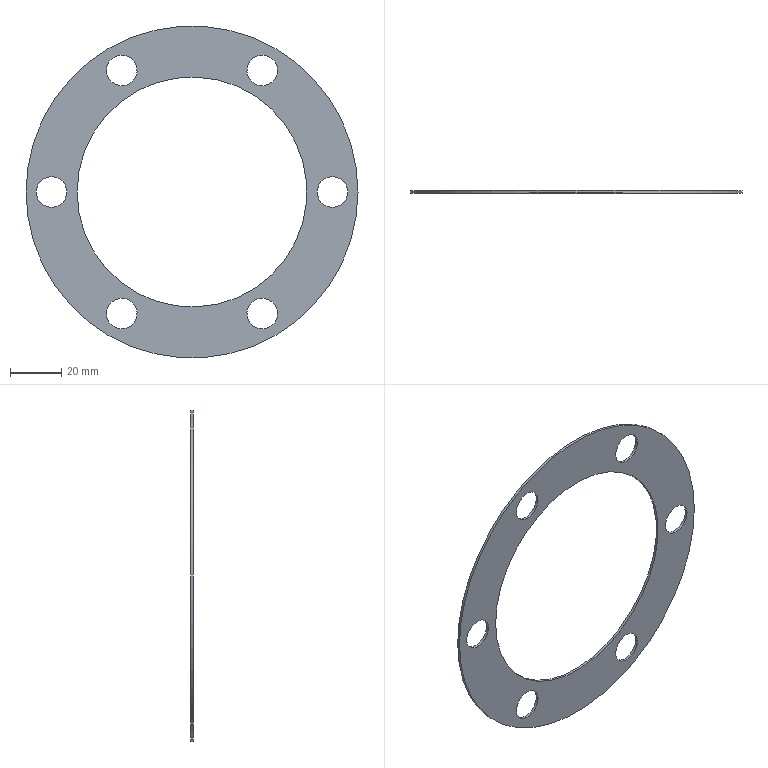Component | NX | T1_SHIM1 | 1 solid | 10 faces | box 130 x 1 x 130 mm | volume 6233 mm3 | cylinder 8 | plane 2 | commonest cylinder face diameters 12 x6 90 x1 130 x1
STEP:
#1=CARTESIAN_POINT('',(0.,0.,0.));
#2=DIRECTION('',(0.,0.,1.));
#3=DIRECTION('',(1.,0.,0.));
#4=AXIS2_PLACEMENT_3D('',#1,#2,#3);
#5=CARTESIAN_POINT('',(-40.,-81.,113.5));
#6=VERTEX_POINT('',#5);
#7=CARTESIAN_POINT('',(5.,-81.,113.5));
#8=DIRECTION('',(0.,1.,0.));
#9=DIRECTION('',(-1.,0.,0.));
#10=AXIS2_PLACEMENT_3D('',#7,#8,#9);
#11=CIRCLE('',#10,45.);
#12=CARTESIAN_POINT('',(5.,-81.,113.5));
#13=DIRECTION('',(0.,-1.,0.));
#14=DIRECTION('',(1.,0.,0.));
#15=AXIS2_PLACEMENT_3D('',#12,#13,#14);
#16=CYLINDRICAL_SURFACE('',#15,45.);
#17=CARTESIAN_POINT('',(9.425,0.));
#18=DIRECTION('',(-1.,0.));
#19=VECTOR('',#18,1.);
#20=LINE('',#17,#19);
#21=(GEOMETRIC_REPRESENTATION_CONTEXT(2)PARAMETRIC_REPRESENTATION_CONTEXT()REPRESENTATION_CONTEXT('',''));
#22=DEFINITIONAL_REPRESENTATION('',(#20),#21);
#23=PCURVE('',#16,#22);
#24=CARTESIAN_POINT('',(-22.5,-81.,113.5));
#25=DIRECTION('',(0.,1.,0.));
#26=DIRECTION('',(-1.,0.,0.));
#27=AXIS2_PLACEMENT_3D('',#24,#25,#26);
#28=PLANE('',#27);
#29=CARTESIAN_POINT('',(-27.5,0.));
#30=DIRECTION('',(1.,0.));
#31=AXIS2_PLACEMENT_2D('',#29,#30);
#32=CIRCLE('',#31,45.);
#33=(GEOMETRIC_REPRESENTATION_CONTEXT(2)PARAMETRIC_REPRESENTATION_CONTEXT()REPRESENTATION_CONTEXT('',''));
#34=DEFINITIONAL_REPRESENTATION('',(#32),#33);
#35=PCURVE('',#28,#34);
#36=SURFACE_CURVE('',#11,(#23,#35),.PCURVE_S1.);
#37=EDGE_CURVE('',#6,#6,#36,.T.);
#38=ORIENTED_EDGE('',*,*,#37,.F.);
#39=CARTESIAN_POINT('',(-40.,-82.,113.5));
#40=VERTEX_POINT('',#39);
#41=CARTESIAN_POINT('',(-40.,-81.,113.5));
#42=CARTESIAN_POINT('',(-40.,-82.,113.5));
#43=B_SPLINE_CURVE_WITH_KNOTS('',1,(#41,#42),.UNSPECIFIED.,.F.,.F.,(2,2),(0.,1.),.PIECEWISE_BEZIER_KNOTS.);
#44=CARTESIAN_POINT('',(9.425,0.));
#45=DIRECTION('',(0.,1.));
#46=VECTOR('',#45,1.);
#47=LINE('',#44,#46);
#48=(GEOMETRIC_REPRESENTATION_CONTEXT(2)PARAMETRIC_REPRESENTATION_CONTEXT()REPRESENTATION_CONTEXT('',''));
#49=DEFINITIONAL_REPRESENTATION('',(#47),#48);
#50=PCURVE('',#16,#49);
#51=CARTESIAN_POINT('',(3.142,0.));
#52=DIRECTION('',(0.,1.));
#53=VECTOR('',#52,1.);
#54=LINE('',#51,#53);
#55=(GEOMETRIC_REPRESENTATION_CONTEXT(2)PARAMETRIC_REPRESENTATION_CONTEXT()REPRESENTATION_CONTEXT('',''));
#56=DEFINITIONAL_REPRESENTATION('',(#54),#55);
#57=PCURVE('',#16,#56);
#58=SEAM_CURVE('',#43,(#50,#57),.PCURVE_S1.);
#59=EDGE_CURVE('',#6,#40,#58,.T.);
#60=ORIENTED_EDGE('',*,*,#59,.T.);
#61=CARTESIAN_POINT('',(5.,-82.,113.5));
#62=DIRECTION('',(0.,1.,0.));
#63=DIRECTION('',(-1.,0.,0.));
#64=AXIS2_PLACEMENT_3D('',#61,#62,#63);
#65=CIRCLE('',#64,45.);
#66=CARTESIAN_POINT('',(9.425,1.));
#67=DIRECTION('',(-1.,0.));
#68=VECTOR('',#67,1.);
#69=LINE('',#66,#68);
#70=(GEOMETRIC_REPRESENTATION_CONTEXT(2)PARAMETRIC_REPRESENTATION_CONTEXT()REPRESENTATION_CONTEXT('',''));
#71=DEFINITIONAL_REPRESENTATION('',(#69),#70);
#72=PCURVE('',#16,#71);
#73=CARTESIAN_POINT('',(-22.5,-82.,113.5));
#74=DIRECTION('',(0.,1.,0.));
#75=DIRECTION('',(-1.,0.,0.));
#76=AXIS2_PLACEMENT_3D('',#73,#74,#75);
#77=PLANE('',#76);
#78=CARTESIAN_POINT('',(-27.5,0.));
#79=DIRECTION('',(1.,0.));
#80=AXIS2_PLACEMENT_2D('',#78,#79);
#81=CIRCLE('',#80,45.);
#82=(GEOMETRIC_REPRESENTATION_CONTEXT(2)PARAMETRIC_REPRESENTATION_CONTEXT()REPRESENTATION_CONTEXT('',''));
#83=DEFINITIONAL_REPRESENTATION('',(#81),#82);
#84=PCURVE('',#77,#83);
#85=SURFACE_CURVE('',#65,(#72,#84),.PCURVE_S1.);
#86=EDGE_CURVE('',#40,#40,#85,.T.);
#87=ORIENTED_EDGE('',*,*,#86,.T.);
#88=ORIENTED_EDGE('',*,*,#59,.F.);
#89=EDGE_LOOP('',(#38,#60,#87,#88));
#90=FACE_BOUND('',#89,.F.);
#91=ADVANCED_FACE('',(#90),#16,.F.);
#92=CARTESIAN_POINT('',(35.5,-81.,60.672));
#93=VERTEX_POINT('',#92);
#94=CARTESIAN_POINT('',(32.5,-81.,65.869));
#95=DIRECTION('',(0.,1.,0.));
#96=DIRECTION('',(0.5,0.,-0.866));
#97=AXIS2_PLACEMENT_3D('',#94,#95,#96);
#98=CIRCLE('',#97,6.);
#99=CARTESIAN_POINT('',(32.5,-81.,65.869));
#100=DIRECTION('',(0.,-1.,0.));
#101=DIRECTION('',(1.,0.,0.));
#102=AXIS2_PLACEMENT_3D('',#99,#100,#101);
#103=CYLINDRICAL_SURFACE('',#102,6.);
#104=CARTESIAN_POINT('',(11.519,0.));
#105=DIRECTION('',(-1.,0.));
#106=VECTOR('',#105,1.);
#107=LINE('',#104,#106);
#108=(GEOMETRIC_REPRESENTATION_CONTEXT(2)PARAMETRIC_REPRESENTATION_CONTEXT()REPRESENTATION_CONTEXT('',''));
#109=DEFINITIONAL_REPRESENTATION('',(#107),#108);
#110=PCURVE('',#103,#109);
#111=CARTESIAN_POINT('',(-55.,-47.631));
#112=DIRECTION('',(-0.5,-0.866));
#113=AXIS2_PLACEMENT_2D('',#111,#112);
#114=CIRCLE('',#113,6.);
#115=(GEOMETRIC_REPRESENTATION_CONTEXT(2)PARAMETRIC_REPRESENTATION_CONTEXT()REPRESENTATION_CONTEXT('',''));
#116=DEFINITIONAL_REPRESENTATION('',(#114),#115);
#117=PCURVE('',#28,#116);
#118=SURFACE_CURVE('',#98,(#110,#117),.PCURVE_S1.);
#119=EDGE_CURVE('',#93,#93,#118,.T.);
#120=ORIENTED_EDGE('',*,*,#119,.F.);
#121=CARTESIAN_POINT('',(35.5,-82.,60.672));
#122=VERTEX_POINT('',#121);
#123=CARTESIAN_POINT('',(35.5,-81.,60.672));
#124=CARTESIAN_POINT('',(35.5,-82.,60.672));
#125=B_SPLINE_CURVE_WITH_KNOTS('',1,(#123,#124),.UNSPECIFIED.,.F.,.F.,(2,2),(0.,1.),.PIECEWISE_BEZIER_KNOTS.);
#126=CARTESIAN_POINT('',(11.519,0.));
#127=DIRECTION('',(0.,1.));
#128=VECTOR('',#127,1.);
#129=LINE('',#126,#128);
#130=(GEOMETRIC_REPRESENTATION_CONTEXT(2)PARAMETRIC_REPRESENTATION_CONTEXT()REPRESENTATION_CONTEXT('',''));
#131=DEFINITIONAL_REPRESENTATION('',(#129),#130);
#132=PCURVE('',#103,#131);
#133=CARTESIAN_POINT('',(5.236,0.));
#134=DIRECTION('',(0.,1.));
#135=VECTOR('',#134,1.);
#136=LINE('',#133,#135);
#137=(GEOMETRIC_REPRESENTATION_CONTEXT(2)PARAMETRIC_REPRESENTATION_CONTEXT()REPRESENTATION_CONTEXT('',''));
#138=DEFINITIONAL_REPRESENTATION('',(#136),#137);
#139=PCURVE('',#103,#138);
#140=SEAM_CURVE('',#125,(#132,#139),.PCURVE_S1.);
#141=EDGE_CURVE('',#93,#122,#140,.T.);
#142=ORIENTED_EDGE('',*,*,#141,.T.);
#143=CARTESIAN_POINT('',(32.5,-82.,65.869));
#144=DIRECTION('',(0.,1.,0.));
#145=DIRECTION('',(0.5,0.,-0.866));
#146=AXIS2_PLACEMENT_3D('',#143,#144,#145);
#147=CIRCLE('',#146,6.);
#148=CARTESIAN_POINT('',(11.519,1.));
#149=DIRECTION('',(-1.,0.));
#150=VECTOR('',#149,1.);
#151=LINE('',#148,#150);
#152=(GEOMETRIC_REPRESENTATION_CONTEXT(2)PARAMETRIC_REPRESENTATION_CONTEXT()REPRESENTATION_CONTEXT('',''));
#153=DEFINITIONAL_REPRESENTATION('',(#151),#152);
#154=PCURVE('',#103,#153);
#155=CARTESIAN_POINT('',(-55.,-47.631));
#156=DIRECTION('',(-0.5,-0.866));
#157=AXIS2_PLACEMENT_2D('',#155,#156);
#158=CIRCLE('',#157,6.);
#159=(GEOMETRIC_REPRESENTATION_CONTEXT(2)PARAMETRIC_REPRESENTATION_CONTEXT()REPRESENTATION_CONTEXT('',''));
#160=DEFINITIONAL_REPRESENTATION('',(#158),#159);
#161=PCURVE('',#77,#160);
#162=SURFACE_CURVE('',#147,(#154,#161),.PCURVE_S1.);
#163=EDGE_CURVE('',#122,#122,#162,.T.);
#164=ORIENTED_EDGE('',*,*,#163,.T.);
#165=ORIENTED_EDGE('',*,*,#141,.F.);
#166=EDGE_LOOP('',(#120,#142,#164,#165));
#167=FACE_BOUND('',#166,.F.);
#168=ADVANCED_FACE('',(#167),#103,.F.);
#169=CARTESIAN_POINT('',(35.5,-81.,166.328));
#170=VERTEX_POINT('',#169);
#171=CARTESIAN_POINT('',(32.5,-81.,161.131));
#172=DIRECTION('',(0.,1.,0.));
#173=DIRECTION('',(0.5,0.,0.866));
#174=AXIS2_PLACEMENT_3D('',#171,#172,#173);
#175=CIRCLE('',#174,6.);
#176=CARTESIAN_POINT('',(32.5,-81.,161.131));
#177=DIRECTION('',(0.,-1.,0.));
#178=DIRECTION('',(1.,0.,0.));
#179=AXIS2_PLACEMENT_3D('',#176,#177,#178);
#180=CYLINDRICAL_SURFACE('',#179,6.);
#181=CARTESIAN_POINT('',(7.33,0.));
#182=DIRECTION('',(-1.,0.));
#183=VECTOR('',#182,1.);
#184=LINE('',#181,#183);
#185=(GEOMETRIC_REPRESENTATION_CONTEXT(2)PARAMETRIC_REPRESENTATION_CONTEXT()REPRESENTATION_CONTEXT('',''));
#186=DEFINITIONAL_REPRESENTATION('',(#184),#185);
#187=PCURVE('',#180,#186);
#188=CARTESIAN_POINT('',(-55.,47.631));
#189=DIRECTION('',(-0.5,0.866));
#190=AXIS2_PLACEMENT_2D('',#188,#189);
#191=CIRCLE('',#190,6.);
#192=(GEOMETRIC_REPRESENTATION_CONTEXT(2)PARAMETRIC_REPRESENTATION_CONTEXT()REPRESENTATION_CONTEXT('',''));
#193=DEFINITIONAL_REPRESENTATION('',(#191),#192);
#194=PCURVE('',#28,#193);
#195=SURFACE_CURVE('',#175,(#187,#194),.PCURVE_S1.);
#196=EDGE_CURVE('',#170,#170,#195,.T.);
#197=ORIENTED_EDGE('',*,*,#196,.F.);
#198=CARTESIAN_POINT('',(35.5,-82.,166.328));
#199=VERTEX_POINT('',#198);
#200=CARTESIAN_POINT('',(35.5,-81.,166.328));
#201=CARTESIAN_POINT('',(35.5,-82.,166.328));
#202=B_SPLINE_CURVE_WITH_KNOTS('',1,(#200,#201),.UNSPECIFIED.,.F.,.F.,(2,2),(0.,1.),.PIECEWISE_BEZIER_KNOTS.);
#203=CARTESIAN_POINT('',(7.33,0.));
#204=DIRECTION('',(0.,1.));
#205=VECTOR('',#204,1.);
#206=LINE('',#203,#205);
#207=(GEOMETRIC_REPRESENTATION_CONTEXT(2)PARAMETRIC_REPRESENTATION_CONTEXT()REPRESENTATION_CONTEXT('',''));
#208=DEFINITIONAL_REPRESENTATION('',(#206),#207);
#209=PCURVE('',#180,#208);
#210=CARTESIAN_POINT('',(1.047,0.));
#211=DIRECTION('',(0.,1.));
#212=VECTOR('',#211,1.);
#213=LINE('',#210,#212);
#214=(GEOMETRIC_REPRESENTATION_CONTEXT(2)PARAMETRIC_REPRESENTATION_CONTEXT()REPRESENTATION_CONTEXT('',''));
#215=DEFINITIONAL_REPRESENTATION('',(#213),#214);
#216=PCURVE('',#180,#215);
#217=SEAM_CURVE('',#202,(#209,#216),.PCURVE_S1.);
#218=EDGE_CURVE('',#170,#199,#217,.T.);
#219=ORIENTED_EDGE('',*,*,#218,.T.);
#220=CARTESIAN_POINT('',(32.5,-82.,161.131));
#221=DIRECTION('',(0.,1.,0.));
#222=DIRECTION('',(0.5,0.,0.866));
#223=AXIS2_PLACEMENT_3D('',#220,#221,#222);
#224=CIRCLE('',#223,6.);
#225=CARTESIAN_POINT('',(7.33,1.));
#226=DIRECTION('',(-1.,0.));
#227=VECTOR('',#226,1.);
#228=LINE('',#225,#227);
#229=(GEOMETRIC_REPRESENTATION_CONTEXT(2)PARAMETRIC_REPRESENTATION_CONTEXT()REPRESENTATION_CONTEXT('',''));
#230=DEFINITIONAL_REPRESENTATION('',(#228),#229);
#231=PCURVE('',#180,#230);
#232=CARTESIAN_POINT('',(-55.,47.631));
#233=DIRECTION('',(-0.5,0.866));
#234=AXIS2_PLACEMENT_2D('',#232,#233);
#235=CIRCLE('',#234,6.);
#236=(GEOMETRIC_REPRESENTATION_CONTEXT(2)PARAMETRIC_REPRESENTATION_CONTEXT()REPRESENTATION_CONTEXT('',''));
#237=DEFINITIONAL_REPRESENTATION('',(#235),#236);
#238=PCURVE('',#77,#237);
#239=SURFACE_CURVE('',#224,(#231,#238),.PCURVE_S1.);
#240=EDGE_CURVE('',#199,#199,#239,.T.);
#241=ORIENTED_EDGE('',*,*,#240,.T.);
#242=ORIENTED_EDGE('',*,*,#218,.F.);
#243=EDGE_LOOP('',(#197,#219,#241,#242));
#244=FACE_BOUND('',#243,.F.);
#245=ADVANCED_FACE('',(#244),#180,.F.);
#246=CARTESIAN_POINT('',(-25.5,-81.,60.672));
#247=VERTEX_POINT('',#246);
#248=CARTESIAN_POINT('',(-22.5,-81.,65.869));
#249=DIRECTION('',(0.,1.,0.));
#250=DIRECTION('',(-0.5,0.,-0.866));
#251=AXIS2_PLACEMENT_3D('',#248,#249,#250);
#252=CIRCLE('',#251,6.);
#253=CARTESIAN_POINT('',(-22.5,-81.,65.869));
#254=DIRECTION('',(0.,-1.,0.));
#255=DIRECTION('',(1.,0.,0.));
#256=AXIS2_PLACEMENT_3D('',#253,#254,#255);
#257=CYLINDRICAL_SURFACE('',#256,6.);
#258=CARTESIAN_POINT('',(10.472,0.));
#259=DIRECTION('',(-1.,0.));
#260=VECTOR('',#259,1.);
#261=LINE('',#258,#260);
#262=(GEOMETRIC_REPRESENTATION_CONTEXT(2)PARAMETRIC_REPRESENTATION_CONTEXT()REPRESENTATION_CONTEXT('',''));
#263=DEFINITIONAL_REPRESENTATION('',(#261),#262);
#264=PCURVE('',#257,#263);
#265=CARTESIAN_POINT('',(-0.,-47.631));
#266=DIRECTION('',(0.5,-0.866));
#267=AXIS2_PLACEMENT_2D('',#265,#266);
#268=CIRCLE('',#267,6.);
#269=(GEOMETRIC_REPRESENTATION_CONTEXT(2)PARAMETRIC_REPRESENTATION_CONTEXT()REPRESENTATION_CONTEXT('',''));
#270=DEFINITIONAL_REPRESENTATION('',(#268),#269);
#271=PCURVE('',#28,#270);
#272=SURFACE_CURVE('',#252,(#264,#271),.PCURVE_S1.);
#273=EDGE_CURVE('',#247,#247,#272,.T.);
#274=ORIENTED_EDGE('',*,*,#273,.F.);
#275=CARTESIAN_POINT('',(-25.5,-82.,60.672));
#276=VERTEX_POINT('',#275);
#277=CARTESIAN_POINT('',(-25.5,-81.,60.672));
#278=CARTESIAN_POINT('',(-25.5,-82.,60.672));
#279=B_SPLINE_CURVE_WITH_KNOTS('',1,(#277,#278),.UNSPECIFIED.,.F.,.F.,(2,2),(0.,1.),.PIECEWISE_BEZIER_KNOTS.);
#280=CARTESIAN_POINT('',(10.472,0.));
#281=DIRECTION('',(0.,1.));
#282=VECTOR('',#281,1.);
#283=LINE('',#280,#282);
#284=(GEOMETRIC_REPRESENTATION_CONTEXT(2)PARAMETRIC_REPRESENTATION_CONTEXT()REPRESENTATION_CONTEXT('',''));
#285=DEFINITIONAL_REPRESENTATION('',(#283),#284);
#286=PCURVE('',#257,#285);
#287=CARTESIAN_POINT('',(4.189,0.));
#288=DIRECTION('',(0.,1.));
#289=VECTOR('',#288,1.);
#290=LINE('',#287,#289);
#291=(GEOMETRIC_REPRESENTATION_CONTEXT(2)PARAMETRIC_REPRESENTATION_CONTEXT()REPRESENTATION_CONTEXT('',''));
#292=DEFINITIONAL_REPRESENTATION('',(#290),#291);
#293=PCURVE('',#257,#292);
#294=SEAM_CURVE('',#279,(#286,#293),.PCURVE_S1.);
#295=EDGE_CURVE('',#247,#276,#294,.T.);
#296=ORIENTED_EDGE('',*,*,#295,.T.);
#297=CARTESIAN_POINT('',(-22.5,-82.,65.869));
#298=DIRECTION('',(0.,1.,0.));
#299=DIRECTION('',(-0.5,0.,-0.866));
#300=AXIS2_PLACEMENT_3D('',#297,#298,#299);
#301=CIRCLE('',#300,6.);
#302=CARTESIAN_POINT('',(10.472,1.));
#303=DIRECTION('',(-1.,0.));
#304=VECTOR('',#303,1.);
#305=LINE('',#302,#304);
#306=(GEOMETRIC_REPRESENTATION_CONTEXT(2)PARAMETRIC_REPRESENTATION_CONTEXT()REPRESENTATION_CONTEXT('',''));
#307=DEFINITIONAL_REPRESENTATION('',(#305),#306);
#308=PCURVE('',#257,#307);
#309=CARTESIAN_POINT('',(-0.,-47.631));
#310=DIRECTION('',(0.5,-0.866));
#311=AXIS2_PLACEMENT_2D('',#309,#310);
#312=CIRCLE('',#311,6.);
#313=(GEOMETRIC_REPRESENTATION_CONTEXT(2)PARAMETRIC_REPRESENTATION_CONTEXT()REPRESENTATION_CONTEXT('',''));
#314=DEFINITIONAL_REPRESENTATION('',(#312),#313);
#315=PCURVE('',#77,#314);
#316=SURFACE_CURVE('',#301,(#308,#315),.PCURVE_S1.);
#317=EDGE_CURVE('',#276,#276,#316,.T.);
#318=ORIENTED_EDGE('',*,*,#317,.T.);
#319=ORIENTED_EDGE('',*,*,#295,.F.);
#320=EDGE_LOOP('',(#274,#296,#318,#319));
#321=FACE_BOUND('',#320,.F.);
#322=ADVANCED_FACE('',(#321),#257,.F.);
#323=CARTESIAN_POINT('',(-25.5,-81.,166.328));
#324=VERTEX_POINT('',#323);
#325=CARTESIAN_POINT('',(-22.5,-81.,161.131));
#326=DIRECTION('',(0.,1.,0.));
#327=DIRECTION('',(-0.5,0.,0.866));
#328=AXIS2_PLACEMENT_3D('',#325,#326,#327);
#329=CIRCLE('',#328,6.);
#330=CARTESIAN_POINT('',(-22.5,-81.,161.131));
#331=DIRECTION('',(0.,-1.,0.));
#332=DIRECTION('',(1.,0.,0.));
#333=AXIS2_PLACEMENT_3D('',#330,#331,#332);
#334=CYLINDRICAL_SURFACE('',#333,6.);
#335=CARTESIAN_POINT('',(8.378,0.));
#336=DIRECTION('',(-1.,0.));
#337=VECTOR('',#336,1.);
#338=LINE('',#335,#337);
#339=(GEOMETRIC_REPRESENTATION_CONTEXT(2)PARAMETRIC_REPRESENTATION_CONTEXT()REPRESENTATION_CONTEXT('',''));
#340=DEFINITIONAL_REPRESENTATION('',(#338),#339);
#341=PCURVE('',#334,#340);
#342=CARTESIAN_POINT('',(0.,47.631));
#343=DIRECTION('',(0.5,0.866));
#344=AXIS2_PLACEMENT_2D('',#342,#343);
#345=CIRCLE('',#344,6.);
#346=(GEOMETRIC_REPRESENTATION_CONTEXT(2)PARAMETRIC_REPRESENTATION_CONTEXT()REPRESENTATION_CONTEXT('',''));
#347=DEFINITIONAL_REPRESENTATION('',(#345),#346);
#348=PCURVE('',#28,#347);
#349=SURFACE_CURVE('',#329,(#341,#348),.PCURVE_S1.);
#350=EDGE_CURVE('',#324,#324,#349,.T.);
#351=ORIENTED_EDGE('',*,*,#350,.F.);
#352=CARTESIAN_POINT('',(-25.5,-82.,166.328));
#353=VERTEX_POINT('',#352);
#354=CARTESIAN_POINT('',(-25.5,-81.,166.328));
#355=CARTESIAN_POINT('',(-25.5,-82.,166.328));
#356=B_SPLINE_CURVE_WITH_KNOTS('',1,(#354,#355),.UNSPECIFIED.,.F.,.F.,(2,2),(0.,1.),.PIECEWISE_BEZIER_KNOTS.);
#357=CARTESIAN_POINT('',(8.378,0.));
#358=DIRECTION('',(0.,1.));
#359=VECTOR('',#358,1.);
#360=LINE('',#357,#359);
#361=(GEOMETRIC_REPRESENTATION_CONTEXT(2)PARAMETRIC_REPRESENTATION_CONTEXT()REPRESENTATION_CONTEXT('',''));
#362=DEFINITIONAL_REPRESENTATION('',(#360),#361);
#363=PCURVE('',#334,#362);
#364=CARTESIAN_POINT('',(2.094,0.));
#365=DIRECTION('',(0.,1.));
#366=VECTOR('',#365,1.);
#367=LINE('',#364,#366);
#368=(GEOMETRIC_REPRESENTATION_CONTEXT(2)PARAMETRIC_REPRESENTATION_CONTEXT()REPRESENTATION_CONTEXT('',''));
#369=DEFINITIONAL_REPRESENTATION('',(#367),#368);
#370=PCURVE('',#334,#369);
#371=SEAM_CURVE('',#356,(#363,#370),.PCURVE_S1.);
#372=EDGE_CURVE('',#324,#353,#371,.T.);
#373=ORIENTED_EDGE('',*,*,#372,.T.);
#374=CARTESIAN_POINT('',(-22.5,-82.,161.131));
#375=DIRECTION('',(0.,1.,0.));
#376=DIRECTION('',(-0.5,0.,0.866));
#377=AXIS2_PLACEMENT_3D('',#374,#375,#376);
#378=CIRCLE('',#377,6.);
#379=CARTESIAN_POINT('',(8.378,1.));
#380=DIRECTION('',(-1.,0.));
#381=VECTOR('',#380,1.);
#382=LINE('',#379,#381);
#383=(GEOMETRIC_REPRESENTATION_CONTEXT(2)PARAMETRIC_REPRESENTATION_CONTEXT()REPRESENTATION_CONTEXT('',''));
#384=DEFINITIONAL_REPRESENTATION('',(#382),#383);
#385=PCURVE('',#334,#384);
#386=CARTESIAN_POINT('',(0.,47.631));
#387=DIRECTION('',(0.5,0.866));
#388=AXIS2_PLACEMENT_2D('',#386,#387);
#389=CIRCLE('',#388,6.);
#390=(GEOMETRIC_REPRESENTATION_CONTEXT(2)PARAMETRIC_REPRESENTATION_CONTEXT()REPRESENTATION_CONTEXT('',''));
#391=DEFINITIONAL_REPRESENTATION('',(#389),#390);
#392=PCURVE('',#77,#391);
#393=SURFACE_CURVE('',#378,(#385,#392),.PCURVE_S1.);
#394=EDGE_CURVE('',#353,#353,#393,.T.);
#395=ORIENTED_EDGE('',*,*,#394,.T.);
#396=ORIENTED_EDGE('',*,*,#372,.F.);
#397=EDGE_LOOP('',(#351,#373,#395,#396));
#398=FACE_BOUND('',#397,.F.);
#399=ADVANCED_FACE('',(#398),#334,.F.);
#400=CARTESIAN_POINT('',(-56.,-81.,113.5));
#401=VERTEX_POINT('',#400);
#402=CARTESIAN_POINT('',(-50.,-81.,113.5));
#403=DIRECTION('',(0.,1.,0.));
#404=DIRECTION('',(-1.,0.,0.));
#405=AXIS2_PLACEMENT_3D('',#402,#403,#404);
#406=CIRCLE('',#405,6.);
#407=CARTESIAN_POINT('',(-50.,-81.,113.5));
#408=DIRECTION('',(0.,-1.,0.));
#409=DIRECTION('',(1.,0.,0.));
#410=AXIS2_PLACEMENT_3D('',#407,#408,#409);
#411=CYLINDRICAL_SURFACE('',#410,6.);
#412=CARTESIAN_POINT('',(9.425,0.));
#413=DIRECTION('',(-1.,0.));
#414=VECTOR('',#413,1.);
#415=LINE('',#412,#414);
#416=(GEOMETRIC_REPRESENTATION_CONTEXT(2)PARAMETRIC_REPRESENTATION_CONTEXT()REPRESENTATION_CONTEXT('',''));
#417=DEFINITIONAL_REPRESENTATION('',(#415),#416);
#418=PCURVE('',#411,#417);
#419=CARTESIAN_POINT('',(27.5,0.));
#420=DIRECTION('',(1.,0.));
#421=AXIS2_PLACEMENT_2D('',#419,#420);
#422=CIRCLE('',#421,6.);
#423=(GEOMETRIC_REPRESENTATION_CONTEXT(2)PARAMETRIC_REPRESENTATION_CONTEXT()REPRESENTATION_CONTEXT('',''));
#424=DEFINITIONAL_REPRESENTATION('',(#422),#423);
#425=PCURVE('',#28,#424);
#426=SURFACE_CURVE('',#406,(#418,#425),.PCURVE_S1.);
#427=EDGE_CURVE('',#401,#401,#426,.T.);
#428=ORIENTED_EDGE('',*,*,#427,.F.);
#429=CARTESIAN_POINT('',(-56.,-82.,113.5));
#430=VERTEX_POINT('',#429);
#431=CARTESIAN_POINT('',(-56.,-81.,113.5));
#432=CARTESIAN_POINT('',(-56.,-82.,113.5));
#433=B_SPLINE_CURVE_WITH_KNOTS('',1,(#431,#432),.UNSPECIFIED.,.F.,.F.,(2,2),(0.,1.),.PIECEWISE_BEZIER_KNOTS.);
#434=CARTESIAN_POINT('',(9.425,0.));
#435=DIRECTION('',(0.,1.));
#436=VECTOR('',#435,1.);
#437=LINE('',#434,#436);
#438=(GEOMETRIC_REPRESENTATION_CONTEXT(2)PARAMETRIC_REPRESENTATION_CONTEXT()REPRESENTATION_CONTEXT('',''));
#439=DEFINITIONAL_REPRESENTATION('',(#437),#438);
#440=PCURVE('',#411,#439);
#441=CARTESIAN_POINT('',(3.142,0.));
#442=DIRECTION('',(0.,1.));
#443=VECTOR('',#442,1.);
#444=LINE('',#441,#443);
#445=(GEOMETRIC_REPRESENTATION_CONTEXT(2)PARAMETRIC_REPRESENTATION_CONTEXT()REPRESENTATION_CONTEXT('',''));
#446=DEFINITIONAL_REPRESENTATION('',(#444),#445);
#447=PCURVE('',#411,#446);
#448=SEAM_CURVE('',#433,(#440,#447),.PCURVE_S1.);
#449=EDGE_CURVE('',#401,#430,#448,.T.);
#450=ORIENTED_EDGE('',*,*,#449,.T.);
#451=CARTESIAN_POINT('',(-50.,-82.,113.5));
#452=DIRECTION('',(0.,1.,0.));
#453=DIRECTION('',(-1.,0.,0.));
#454=AXIS2_PLACEMENT_3D('',#451,#452,#453);
#455=CIRCLE('',#454,6.);
#456=CARTESIAN_POINT('',(9.425,1.));
#457=DIRECTION('',(-1.,0.));
#458=VECTOR('',#457,1.);
#459=LINE('',#456,#458);
#460=(GEOMETRIC_REPRESENTATION_CONTEXT(2)PARAMETRIC_REPRESENTATION_CONTEXT()REPRESENTATION_CONTEXT('',''));
#461=DEFINITIONAL_REPRESENTATION('',(#459),#460);
#462=PCURVE('',#411,#461);
#463=CARTESIAN_POINT('',(27.5,0.));
#464=DIRECTION('',(1.,0.));
#465=AXIS2_PLACEMENT_2D('',#463,#464);
#466=CIRCLE('',#465,6.);
#467=(GEOMETRIC_REPRESENTATION_CONTEXT(2)PARAMETRIC_REPRESENTATION_CONTEXT()REPRESENTATION_CONTEXT('',''));
#468=DEFINITIONAL_REPRESENTATION('',(#466),#467);
#469=PCURVE('',#77,#468);
#470=SURFACE_CURVE('',#455,(#462,#469),.PCURVE_S1.);
#471=EDGE_CURVE('',#430,#430,#470,.T.);
#472=ORIENTED_EDGE('',*,*,#471,.T.);
#473=ORIENTED_EDGE('',*,*,#449,.F.);
#474=EDGE_LOOP('',(#428,#450,#472,#473));
#475=FACE_BOUND('',#474,.F.);
#476=ADVANCED_FACE('',(#475),#411,.F.);
#477=CARTESIAN_POINT('',(-60.,-81.,113.5));
#478=VERTEX_POINT('',#477);
#479=CARTESIAN_POINT('',(5.,-81.,113.5));
#480=DIRECTION('',(0.,1.,0.));
#481=DIRECTION('',(-1.,0.,0.));
#482=AXIS2_PLACEMENT_3D('',#479,#480,#481);
#483=CIRCLE('',#482,65.);
#484=CARTESIAN_POINT('',(5.,-81.,113.5));
#485=DIRECTION('',(0.,-1.,0.));
#486=DIRECTION('',(1.,0.,0.));
#487=AXIS2_PLACEMENT_3D('',#484,#485,#486);
#488=CYLINDRICAL_SURFACE('',#487,65.);
#489=CARTESIAN_POINT('',(9.425,0.));
#490=DIRECTION('',(-1.,0.));
#491=VECTOR('',#490,1.);
#492=LINE('',#489,#491);
#493=(GEOMETRIC_REPRESENTATION_CONTEXT(2)PARAMETRIC_REPRESENTATION_CONTEXT()REPRESENTATION_CONTEXT('',''));
#494=DEFINITIONAL_REPRESENTATION('',(#492),#493);
#495=PCURVE('',#488,#494);
#496=CARTESIAN_POINT('',(-27.5,0.));
#497=DIRECTION('',(1.,0.));
#498=AXIS2_PLACEMENT_2D('',#496,#497);
#499=CIRCLE('',#498,65.);
#500=(GEOMETRIC_REPRESENTATION_CONTEXT(2)PARAMETRIC_REPRESENTATION_CONTEXT()REPRESENTATION_CONTEXT('',''));
#501=DEFINITIONAL_REPRESENTATION('',(#499),#500);
#502=PCURVE('',#28,#501);
#503=SURFACE_CURVE('',#483,(#495,#502),.PCURVE_S1.);
#504=EDGE_CURVE('',#478,#478,#503,.T.);
#505=ORIENTED_EDGE('',*,*,#504,.F.);
#506=CARTESIAN_POINT('',(-60.,-82.,113.5));
#507=VERTEX_POINT('',#506);
#508=CARTESIAN_POINT('',(-60.,-81.,113.5));
#509=CARTESIAN_POINT('',(-60.,-82.,113.5));
#510=B_SPLINE_CURVE_WITH_KNOTS('',1,(#508,#509),.UNSPECIFIED.,.F.,.F.,(2,2),(0.,1.),.PIECEWISE_BEZIER_KNOTS.);
#511=CARTESIAN_POINT('',(9.425,0.));
#512=DIRECTION('',(0.,1.));
#513=VECTOR('',#512,1.);
#514=LINE('',#511,#513);
#515=(GEOMETRIC_REPRESENTATION_CONTEXT(2)PARAMETRIC_REPRESENTATION_CONTEXT()REPRESENTATION_CONTEXT('',''));
#516=DEFINITIONAL_REPRESENTATION('',(#514),#515);
#517=PCURVE('',#488,#516);
#518=CARTESIAN_POINT('',(3.142,0.));
#519=DIRECTION('',(0.,1.));
#520=VECTOR('',#519,1.);
#521=LINE('',#518,#520);
#522=(GEOMETRIC_REPRESENTATION_CONTEXT(2)PARAMETRIC_REPRESENTATION_CONTEXT()REPRESENTATION_CONTEXT('',''));
#523=DEFINITIONAL_REPRESENTATION('',(#521),#522);
#524=PCURVE('',#488,#523);
#525=SEAM_CURVE('',#510,(#517,#524),.PCURVE_S1.);
#526=EDGE_CURVE('',#478,#507,#525,.T.);
#527=ORIENTED_EDGE('',*,*,#526,.T.);
#528=CARTESIAN_POINT('',(5.,-82.,113.5));
#529=DIRECTION('',(0.,1.,0.));
#530=DIRECTION('',(-1.,0.,0.));
#531=AXIS2_PLACEMENT_3D('',#528,#529,#530);
#532=CIRCLE('',#531,65.);
#533=CARTESIAN_POINT('',(9.425,1.));
#534=DIRECTION('',(-1.,0.));
#535=VECTOR('',#534,1.);
#536=LINE('',#533,#535);
#537=(GEOMETRIC_REPRESENTATION_CONTEXT(2)PARAMETRIC_REPRESENTATION_CONTEXT()REPRESENTATION_CONTEXT('',''));
#538=DEFINITIONAL_REPRESENTATION('',(#536),#537);
#539=PCURVE('',#488,#538);
#540=CARTESIAN_POINT('',(-27.5,0.));
#541=DIRECTION('',(1.,0.));
#542=AXIS2_PLACEMENT_2D('',#540,#541);
#543=CIRCLE('',#542,65.);
#544=(GEOMETRIC_REPRESENTATION_CONTEXT(2)PARAMETRIC_REPRESENTATION_CONTEXT()REPRESENTATION_CONTEXT('',''));
#545=DEFINITIONAL_REPRESENTATION('',(#543),#544);
#546=PCURVE('',#77,#545);
#547=SURFACE_CURVE('',#532,(#539,#546),.PCURVE_S1.);
#548=EDGE_CURVE('',#507,#507,#547,.T.);
#549=ORIENTED_EDGE('',*,*,#548,.T.);
#550=ORIENTED_EDGE('',*,*,#526,.F.);
#551=EDGE_LOOP('',(#505,#527,#549,#550));
#552=FACE_BOUND('',#551,.T.);
#553=ADVANCED_FACE('',(#552),#488,.T.);
#554=CARTESIAN_POINT('',(66.,-81.,113.5));
#555=VERTEX_POINT('',#554);
#556=CARTESIAN_POINT('',(60.,-81.,113.5));
#557=DIRECTION('',(0.,1.,0.));
#558=DIRECTION('',(1.,0.,0.));
#559=AXIS2_PLACEMENT_3D('',#556,#557,#558);
#560=CIRCLE('',#559,6.);
#561=CARTESIAN_POINT('',(60.,-81.,113.5));
#562=DIRECTION('',(0.,-1.,0.));
#563=DIRECTION('',(1.,0.,0.));
#564=AXIS2_PLACEMENT_3D('',#561,#562,#563);
#565=CYLINDRICAL_SURFACE('',#564,6.);
#566=CARTESIAN_POINT('',(6.283,0.));
#567=DIRECTION('',(-1.,0.));
#568=VECTOR('',#567,1.);
#569=LINE('',#566,#568);
#570=(GEOMETRIC_REPRESENTATION_CONTEXT(2)PARAMETRIC_REPRESENTATION_CONTEXT()REPRESENTATION_CONTEXT('',''));
#571=DEFINITIONAL_REPRESENTATION('',(#569),#570);
#572=PCURVE('',#565,#571);
#573=CARTESIAN_POINT('',(-82.5,0.));
#574=DIRECTION('',(-1.,0.));
#575=AXIS2_PLACEMENT_2D('',#573,#574);
#576=CIRCLE('',#575,6.);
#577=(GEOMETRIC_REPRESENTATION_CONTEXT(2)PARAMETRIC_REPRESENTATION_CONTEXT()REPRESENTATION_CONTEXT('',''));
#578=DEFINITIONAL_REPRESENTATION('',(#576),#577);
#579=PCURVE('',#28,#578);
#580=SURFACE_CURVE('',#560,(#572,#579),.PCURVE_S1.);
#581=EDGE_CURVE('',#555,#555,#580,.T.);
#582=ORIENTED_EDGE('',*,*,#581,.F.);
#583=CARTESIAN_POINT('',(66.,-82.,113.5));
#584=VERTEX_POINT('',#583);
#585=CARTESIAN_POINT('',(66.,-81.,113.5));
#586=CARTESIAN_POINT('',(66.,-82.,113.5));
#587=B_SPLINE_CURVE_WITH_KNOTS('',1,(#585,#586),.UNSPECIFIED.,.F.,.F.,(2,2),(0.,1.),.PIECEWISE_BEZIER_KNOTS.);
#588=CARTESIAN_POINT('',(6.283,0.));
#589=DIRECTION('',(0.,1.));
#590=VECTOR('',#589,1.);
#591=LINE('',#588,#590);
#592=(GEOMETRIC_REPRESENTATION_CONTEXT(2)PARAMETRIC_REPRESENTATION_CONTEXT()REPRESENTATION_CONTEXT('',''));
#593=DEFINITIONAL_REPRESENTATION('',(#591),#592);
#594=PCURVE('',#565,#593);
#595=CARTESIAN_POINT('',(0.,0.));
#596=DIRECTION('',(0.,1.));
#597=VECTOR('',#596,1.);
#598=LINE('',#595,#597);
#599=(GEOMETRIC_REPRESENTATION_CONTEXT(2)PARAMETRIC_REPRESENTATION_CONTEXT()REPRESENTATION_CONTEXT('',''));
#600=DEFINITIONAL_REPRESENTATION('',(#598),#599);
#601=PCURVE('',#565,#600);
#602=SEAM_CURVE('',#587,(#594,#601),.PCURVE_S1.);
#603=EDGE_CURVE('',#555,#584,#602,.T.);
#604=ORIENTED_EDGE('',*,*,#603,.T.);
#605=CARTESIAN_POINT('',(60.,-82.,113.5));
#606=DIRECTION('',(0.,1.,0.));
#607=DIRECTION('',(1.,0.,0.));
#608=AXIS2_PLACEMENT_3D('',#605,#606,#607);
#609=CIRCLE('',#608,6.);
#610=CARTESIAN_POINT('',(6.283,1.));
#611=DIRECTION('',(-1.,0.));
#612=VECTOR('',#611,1.);
#613=LINE('',#610,#612);
#614=(GEOMETRIC_REPRESENTATION_CONTEXT(2)PARAMETRIC_REPRESENTATION_CONTEXT()REPRESENTATION_CONTEXT('',''));
#615=DEFINITIONAL_REPRESENTATION('',(#613),#614);
#616=PCURVE('',#565,#615);
#617=CARTESIAN_POINT('',(-82.5,0.));
#618=DIRECTION('',(-1.,0.));
#619=AXIS2_PLACEMENT_2D('',#617,#618);
#620=CIRCLE('',#619,6.);
#621=(GEOMETRIC_REPRESENTATION_CONTEXT(2)PARAMETRIC_REPRESENTATION_CONTEXT()REPRESENTATION_CONTEXT('',''));
#622=DEFINITIONAL_REPRESENTATION('',(#620),#621);
#623=PCURVE('',#77,#622);
#624=SURFACE_CURVE('',#609,(#616,#623),.PCURVE_S1.);
#625=EDGE_CURVE('',#584,#584,#624,.T.);
#626=ORIENTED_EDGE('',*,*,#625,.T.);
#627=ORIENTED_EDGE('',*,*,#603,.F.);
#628=EDGE_LOOP('',(#582,#604,#626,#627));
#629=FACE_BOUND('',#628,.F.);
#630=ADVANCED_FACE('',(#629),#565,.F.);
#631=ORIENTED_EDGE('',*,*,#504,.T.);
#632=EDGE_LOOP('',(#631));
#633=FACE_BOUND('',#632,.T.);
#634=ORIENTED_EDGE('',*,*,#427,.F.);
#635=EDGE_LOOP('',(#634));
#636=FACE_BOUND('',#635,.T.);
#637=ORIENTED_EDGE('',*,*,#350,.F.);
#638=EDGE_LOOP('',(#637));
#639=FACE_BOUND('',#638,.T.);
#640=ORIENTED_EDGE('',*,*,#273,.F.);
#641=EDGE_LOOP('',(#640));
#642=FACE_BOUND('',#641,.T.);
#643=ORIENTED_EDGE('',*,*,#196,.F.);
#644=EDGE_LOOP('',(#643));
#645=FACE_BOUND('',#644,.T.);
#646=ORIENTED_EDGE('',*,*,#119,.F.);
#647=EDGE_LOOP('',(#646));
#648=FACE_BOUND('',#647,.T.);
#649=ORIENTED_EDGE('',*,*,#37,.F.);
#650=EDGE_LOOP('',(#649));
#651=FACE_BOUND('',#650,.T.);
#652=ORIENTED_EDGE('',*,*,#581,.F.);
#653=EDGE_LOOP('',(#652));
#654=FACE_BOUND('',#653,.T.);
#655=ADVANCED_FACE('',(#633,#636,#639,#642,#645,#648,#651,#654),#28,.T.);
#656=ORIENTED_EDGE('',*,*,#548,.F.);
#657=EDGE_LOOP('',(#656));
#658=FACE_BOUND('',#657,.T.);
#659=ORIENTED_EDGE('',*,*,#471,.T.);
#660=EDGE_LOOP('',(#659));
#661=FACE_BOUND('',#660,.T.);
#662=ORIENTED_EDGE('',*,*,#394,.T.);
#663=EDGE_LOOP('',(#662));
#664=FACE_BOUND('',#663,.T.);
#665=ORIENTED_EDGE('',*,*,#317,.T.);
#666=EDGE_LOOP('',(#665));
#667=FACE_BOUND('',#666,.T.);
#668=ORIENTED_EDGE('',*,*,#240,.T.);
#669=EDGE_LOOP('',(#668));
#670=FACE_BOUND('',#669,.T.);
#671=ORIENTED_EDGE('',*,*,#163,.T.);
#672=EDGE_LOOP('',(#671));
#673=FACE_BOUND('',#672,.T.);
#674=ORIENTED_EDGE('',*,*,#86,.T.);
#675=EDGE_LOOP('',(#674));
#676=FACE_BOUND('',#675,.T.);
#677=ORIENTED_EDGE('',*,*,#625,.T.);
#678=EDGE_LOOP('',(#677));
#679=FACE_BOUND('',#678,.T.);
#680=ADVANCED_FACE('',(#658,#661,#664,#667,#670,#673,#676,#679),#77,.F.);
#681=CLOSED_SHELL('',(#91,#168,#245,#322,#399,#476,#553,#630,#655,#680));
#682=MANIFOLD_SOLID_BREP('',#681);
#683=(LENGTH_UNIT()NAMED_UNIT(*)SI_UNIT(.MILLI.,.METRE.));
#684=UNCERTAINTY_MEASURE_WITH_UNIT(LENGTH_MEASURE(0.00001),#683,'','');
#685=(NAMED_UNIT(*)PLANE_ANGLE_UNIT()SI_UNIT($,.RADIAN.));
#686=(NAMED_UNIT(*)SI_UNIT($,.STERADIAN.)SOLID_ANGLE_UNIT());
#687=(GEOMETRIC_REPRESENTATION_CONTEXT(3)GLOBAL_UNCERTAINTY_ASSIGNED_CONTEXT((#684))GLOBAL_UNIT_ASSIGNED_CONTEXT((#683,#685,#686))REPRESENTATION_CONTEXT('',''));
#688=ADVANCED_BREP_SHAPE_REPRESENTATION('',(#4,#682),#687);